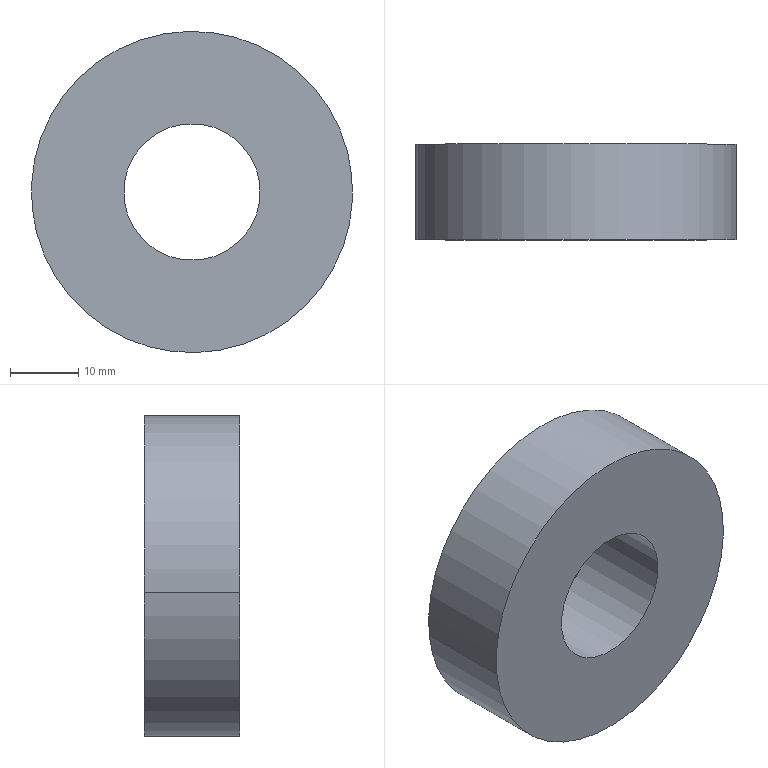Component | SolidWorks | 13-1 | 1 solid | 6 faces | box 47 x 14 x 47 mm | volume 19891 mm3 | cylinder 4 | plane 2 | commonest cylinder face diameters 20 x2 47 x2
build123d program:
from build123d import *

# Parameters (mm, degrees)
SKETCH1_R           = 23.5
SKETCH1_R_2         = 10
BOSS_EXTRUDE1_DEPTH = 14


with BuildPart() as part:
    # Sketch1 → Boss-Extrude1 (new body)
    with BuildSketch(Plane(origin=(0, 0, 0), x_dir=(1, 0, 0), z_dir=(0, 1, 0))):
        with Locations(Location((0, 0, 0), (0, 0, 270))):
            Circle(SKETCH1_R)
        with Locations(Location((0, 0, 0), (0, 0, 270))):
            Circle(SKETCH1_R_2, mode=Mode.SUBTRACT)
    extrude(amount=BOSS_EXTRUDE1_DEPTH)


solid = part.part

# Placed as in the assembly
solid = solid.moved(Location((0, -53.3, 0), (0, 0, 0)))
STEP:
#1=CARTESIAN_POINT('',(0.3916,-1.547,0.04097));
#2=VERTEX_POINT('',#1);
#3=CARTESIAN_POINT('',(-0.3916,-1.547,-0.04097));
#4=VERTEX_POINT('',#3);
#5=CARTESIAN_POINT('',(0.,-1.547,0.));
#6=DIRECTION('',(0.,1.,0.));
#7=DIRECTION('',(-0.9946,0.,-0.1041));
#8=AXIS2_PLACEMENT_3D('',#5,#6,#7);
#9=CIRCLE('',#8,0.3937);
#10=EDGE_CURVE('',#2,#4,#9,.T.);
#11=ORIENTED_EDGE('',*,*,#10,.T.);
#12=CARTESIAN_POINT('',(-0.3916,-2.098,-0.04097));
#13=VERTEX_POINT('',#12);
#14=CARTESIAN_POINT('',(-0.3916,-1.547,-0.04097));
#15=DIRECTION('',(0.,-1.,0.));
#16=VECTOR('',#15,39.37);
#17=LINE('',#14,#16);
#18=EDGE_CURVE('',#4,#13,#17,.T.);
#19=ORIENTED_EDGE('',*,*,#18,.T.);
#20=CARTESIAN_POINT('',(0.3916,-2.098,0.04097));
#21=VERTEX_POINT('',#20);
#22=CARTESIAN_POINT('',(0.,-2.098,0.));
#23=DIRECTION('',(0.,1.,0.));
#24=DIRECTION('',(-0.9946,0.,-0.1041));
#25=AXIS2_PLACEMENT_3D('',#22,#23,#24);
#26=CIRCLE('',#25,0.3937);
#27=EDGE_CURVE('',#21,#13,#26,.T.);
#28=ORIENTED_EDGE('',*,*,#27,.F.);
#29=CARTESIAN_POINT('',(0.3916,-1.547,0.04097));
#30=DIRECTION('',(0.,-1.,0.));
#31=VECTOR('',#30,39.37);
#32=LINE('',#29,#31);
#33=EDGE_CURVE('',#2,#21,#32,.T.);
#34=ORIENTED_EDGE('',*,*,#33,.F.);
#35=EDGE_LOOP('',(#11,#19,#28,#34));
#36=FACE_OUTER_BOUND('',#35,.T.);
#37=CARTESIAN_POINT('',(0.,-1.547,0.));
#38=DIRECTION('',(0.,-1.,0.));
#39=DIRECTION('',(0.9946,0.,0.1041));
#40=AXIS2_PLACEMENT_3D('',#37,#38,#39);
#41=CYLINDRICAL_SURFACE('',#40,0.3937);
#42=ADVANCED_FACE('',(#36),#41,.F.);
#43=CARTESIAN_POINT('',(-0.9202,-1.547,-0.09629));
#44=VERTEX_POINT('',#43);
#45=CARTESIAN_POINT('',(0.9202,-1.547,0.09629));
#46=VERTEX_POINT('',#45);
#47=CARTESIAN_POINT('',(0.,-1.547,0.));
#48=DIRECTION('',(0.,1.,0.));
#49=DIRECTION('',(-0.9946,0.,-0.1041));
#50=AXIS2_PLACEMENT_3D('',#47,#48,#49);
#51=CIRCLE('',#50,0.9252);
#52=EDGE_CURVE('',#44,#46,#51,.T.);
#53=ORIENTED_EDGE('',*,*,#52,.F.);
#54=CARTESIAN_POINT('',(-0.9202,-2.098,-0.09629));
#55=VERTEX_POINT('',#54);
#56=CARTESIAN_POINT('',(-0.9202,-1.547,-0.09629));
#57=DIRECTION('',(0.,-1.,0.));
#58=VECTOR('',#57,39.37);
#59=LINE('',#56,#58);
#60=EDGE_CURVE('',#44,#55,#59,.T.);
#61=ORIENTED_EDGE('',*,*,#60,.T.);
#62=CARTESIAN_POINT('',(0.9202,-2.098,0.09629));
#63=VERTEX_POINT('',#62);
#64=CARTESIAN_POINT('',(0.,-2.098,0.));
#65=DIRECTION('',(0.,1.,0.));
#66=DIRECTION('',(-0.9946,0.,-0.1041));
#67=AXIS2_PLACEMENT_3D('',#64,#65,#66);
#68=CIRCLE('',#67,0.9252);
#69=EDGE_CURVE('',#55,#63,#68,.T.);
#70=ORIENTED_EDGE('',*,*,#69,.T.);
#71=CARTESIAN_POINT('',(0.9202,-1.547,0.09629));
#72=DIRECTION('',(0.,-1.,0.));
#73=VECTOR('',#72,39.37);
#74=LINE('',#71,#73);
#75=EDGE_CURVE('',#46,#63,#74,.T.);
#76=ORIENTED_EDGE('',*,*,#75,.F.);
#77=EDGE_LOOP('',(#53,#61,#70,#76));
#78=FACE_OUTER_BOUND('',#77,.T.);
#79=CARTESIAN_POINT('',(0.,-1.547,0.));
#80=DIRECTION('',(0.,-1.,0.));
#81=DIRECTION('',(0.9946,0.,0.1041));
#82=AXIS2_PLACEMENT_3D('',#79,#80,#81);
#83=CYLINDRICAL_SURFACE('',#82,0.9252);
#84=ADVANCED_FACE('',(#78),#83,.T.);
#85=CARTESIAN_POINT('',(0.,-1.547,0.));
#86=DIRECTION('',(0.,1.,0.));
#87=DIRECTION('',(-0.9946,0.,-0.1041));
#88=AXIS2_PLACEMENT_3D('',#85,#86,#87);
#89=CIRCLE('',#88,0.9252);
#90=EDGE_CURVE('',#46,#44,#89,.T.);
#91=ORIENTED_EDGE('',*,*,#90,.T.);
#92=ORIENTED_EDGE('',*,*,#52,.T.);
#93=EDGE_LOOP('',(#91,#92));
#94=FACE_OUTER_BOUND('',#93,.T.);
#95=ORIENTED_EDGE('',*,*,#10,.F.);
#96=CARTESIAN_POINT('',(0.,-1.547,0.));
#97=DIRECTION('',(0.,1.,0.));
#98=DIRECTION('',(-0.9946,0.,-0.1041));
#99=AXIS2_PLACEMENT_3D('',#96,#97,#98);
#100=CIRCLE('',#99,0.3937);
#101=EDGE_CURVE('',#4,#2,#100,.T.);
#102=ORIENTED_EDGE('',*,*,#101,.F.);
#103=EDGE_LOOP('',(#95,#102));
#104=FACE_BOUND('',#103,.T.);
#105=CARTESIAN_POINT('',(0.,-1.547,0.));
#106=DIRECTION('',(0.,1.,0.));
#107=DIRECTION('',(-0.9946,0.,-0.1041));
#108=AXIS2_PLACEMENT_3D('',#105,#106,#107);
#109=PLANE('',#108);
#110=ADVANCED_FACE('',(#94,#104),#109,.T.);
#111=CARTESIAN_POINT('',(0.,-2.098,0.));
#112=DIRECTION('',(0.,1.,0.));
#113=DIRECTION('',(-0.9946,0.,-0.1041));
#114=AXIS2_PLACEMENT_3D('',#111,#112,#113);
#115=CIRCLE('',#114,0.9252);
#116=EDGE_CURVE('',#63,#55,#115,.T.);
#117=ORIENTED_EDGE('',*,*,#116,.F.);
#118=ORIENTED_EDGE('',*,*,#69,.F.);
#119=EDGE_LOOP('',(#117,#118));
#120=FACE_OUTER_BOUND('',#119,.T.);
#121=ORIENTED_EDGE('',*,*,#27,.T.);
#122=CARTESIAN_POINT('',(0.,-2.098,0.));
#123=DIRECTION('',(0.,1.,0.));
#124=DIRECTION('',(-0.9946,0.,-0.1041));
#125=AXIS2_PLACEMENT_3D('',#122,#123,#124);
#126=CIRCLE('',#125,0.3937);
#127=EDGE_CURVE('',#13,#21,#126,.T.);
#128=ORIENTED_EDGE('',*,*,#127,.T.);
#129=EDGE_LOOP('',(#121,#128));
#130=FACE_BOUND('',#129,.T.);
#131=CARTESIAN_POINT('',(0.,-2.098,0.));
#132=DIRECTION('',(0.,1.,0.));
#133=DIRECTION('',(-0.9946,0.,-0.1041));
#134=AXIS2_PLACEMENT_3D('',#131,#132,#133);
#135=PLANE('',#134);
#136=ADVANCED_FACE('',(#120,#130),#135,.F.);
#137=ORIENTED_EDGE('',*,*,#60,.F.);
#138=ORIENTED_EDGE('',*,*,#90,.F.);
#139=ORIENTED_EDGE('',*,*,#75,.T.);
#140=ORIENTED_EDGE('',*,*,#116,.T.);
#141=EDGE_LOOP('',(#137,#138,#139,#140));
#142=FACE_OUTER_BOUND('',#141,.T.);
#143=CARTESIAN_POINT('',(0.,-1.547,0.));
#144=DIRECTION('',(0.,-1.,0.));
#145=DIRECTION('',(0.9946,0.,0.1041));
#146=AXIS2_PLACEMENT_3D('',#143,#144,#145);
#147=CYLINDRICAL_SURFACE('',#146,0.9252);
#148=ADVANCED_FACE('',(#142),#147,.T.);
#149=ORIENTED_EDGE('',*,*,#18,.F.);
#150=ORIENTED_EDGE('',*,*,#101,.T.);
#151=ORIENTED_EDGE('',*,*,#33,.T.);
#152=ORIENTED_EDGE('',*,*,#127,.F.);
#153=EDGE_LOOP('',(#149,#150,#151,#152));
#154=FACE_OUTER_BOUND('',#153,.T.);
#155=CARTESIAN_POINT('',(0.,-1.547,0.));
#156=DIRECTION('',(0.,-1.,0.));
#157=DIRECTION('',(0.9946,0.,0.1041));
#158=AXIS2_PLACEMENT_3D('',#155,#156,#157);
#159=CYLINDRICAL_SURFACE('',#158,0.3937);
#160=ADVANCED_FACE('',(#154),#159,.F.);
#161=CLOSED_SHELL('',(#42,#84,#110,#136,#148,#160));
#162=MANIFOLD_SOLID_BREP('',#161);
#163=CARTESIAN_POINT('',(0.,0.,0.));
#164=DIRECTION('',(0.,0.,1.));
#165=DIRECTION('',(1.,0.,0.));
#166=AXIS2_PLACEMENT_3D('',#163,#164,#165);
#167=(LENGTH_UNIT()NAMED_UNIT(*)SI_UNIT($,.METRE.));
#168=LENGTH_MEASURE_WITH_UNIT(LENGTH_MEASURE(0.0254),#167);
#169=DIMENSIONAL_EXPONENTS(1.,0.,0.,0.,0.,0.,0.);
#170=(CONVERSION_BASED_UNIT('',#168)LENGTH_UNIT()NAMED_UNIT(#169));
#171=UNCERTAINTY_MEASURE_WITH_UNIT(LENGTH_MEASURE(0.00001),#170,'','');
#172=(NAMED_UNIT(*)PLANE_ANGLE_UNIT()SI_UNIT($,.RADIAN.));
#173=(NAMED_UNIT(*)SI_UNIT($,.STERADIAN.)SOLID_ANGLE_UNIT());
#174=(GEOMETRIC_REPRESENTATION_CONTEXT(3)GLOBAL_UNCERTAINTY_ASSIGNED_CONTEXT((#171))GLOBAL_UNIT_ASSIGNED_CONTEXT((#170,#172,#173))REPRESENTATION_CONTEXT('',''));
#175=ADVANCED_BREP_SHAPE_REPRESENTATION('',(#162,#166),#174);
#176=COLOUR_RGB('',0.7922,0.8196,0.9333);
#177=FILL_AREA_STYLE_COLOUR('',#176);
#178=FILL_AREA_STYLE('',(#177));
#179=SURFACE_STYLE_FILL_AREA(#178);
#180=SURFACE_SIDE_STYLE('',(#179));
#181=SURFACE_STYLE_USAGE(.BOTH.,#180);
#182=PRESENTATION_STYLE_ASSIGNMENT((#181));
#183=STYLED_ITEM('',(#182),#162);
#184=PRESENTATION_LAYER_ASSIGNMENT('','',(#183));
#185=(LENGTH_UNIT()NAMED_UNIT(*)SI_UNIT($,.METRE.));
#186=LENGTH_MEASURE_WITH_UNIT(LENGTH_MEASURE(0.0254),#185);
#187=DIMENSIONAL_EXPONENTS(1.,0.,0.,0.,0.,0.,0.);
#188=(CONVERSION_BASED_UNIT('',#186)LENGTH_UNIT()NAMED_UNIT(#187));
#189=UNCERTAINTY_MEASURE_WITH_UNIT(LENGTH_MEASURE(0.00001),#188,'','');
#190=(NAMED_UNIT(*)PLANE_ANGLE_UNIT()SI_UNIT($,.RADIAN.));
#191=(NAMED_UNIT(*)SI_UNIT($,.STERADIAN.)SOLID_ANGLE_UNIT());
#192=(GEOMETRIC_REPRESENTATION_CONTEXT(3)GLOBAL_UNCERTAINTY_ASSIGNED_CONTEXT((#189))GLOBAL_UNIT_ASSIGNED_CONTEXT((#188,#190,#191))REPRESENTATION_CONTEXT('',''));
#193=MECHANICAL_DESIGN_GEOMETRIC_PRESENTATION_REPRESENTATION('',(#183),#192);